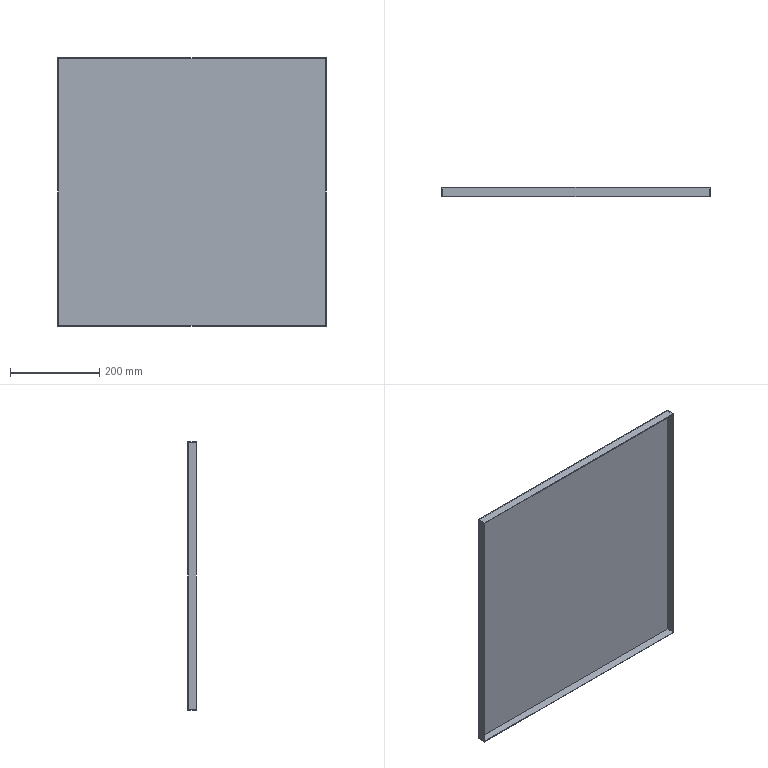Component | SolidWorks | AwningTopPlate-1 | 1 solid | 11 faces | box 600 x 20 x 600 mm | volume 606433 mm3 | plane 11
build123d program:
from build123d import *

# Parameters (mm, degrees)
SKETCH1_W           = 600
SKETCH1_H           = 600
BOSS_EXTRUDE1_DEPTH = 20
SHELL1_T            = -1.5


with BuildPart() as part:
    # Sketch1 → Boss-Extrude1 (new body)
    with BuildSketch(Plane(origin=(0, 0, 0), x_dir=(1, 0, 0), z_dir=(0, 1, 0))):
        Rectangle(SKETCH1_W, SKETCH1_H)
    extrude(amount=BOSS_EXTRUDE1_DEPTH)

    # Shell1
    shell1_openings = [part.faces().sort_by_distance(p)[0] for p in [
        (0, 0, 0),
    ]]
    offset(amount=SHELL1_T, openings=shell1_openings, kind=Kind.INTERSECTION)


solid = part.part

# Placed as in the assembly
solid = solid.moved(Location((0, 1680, 0), (0, 0, 0)))
STEP:
#1=CARTESIAN_POINT('',(11.811,66.142,11.811));
#2=VERTEX_POINT('',#1);
#3=CARTESIAN_POINT('',(11.811,66.142,-11.811));
#4=VERTEX_POINT('',#3);
#5=CARTESIAN_POINT('',(11.811,66.142,-11.811));
#6=DIRECTION('',(0.,0.,-1.));
#7=VECTOR('',#6,39.37);
#8=LINE('',#5,#7);
#9=EDGE_CURVE('',#2,#4,#8,.T.);
#10=ORIENTED_EDGE('',*,*,#9,.T.);
#11=CARTESIAN_POINT('',(11.811,66.929,-11.811));
#12=VERTEX_POINT('',#11);
#13=CARTESIAN_POINT('',(11.811,66.929,-11.811));
#14=DIRECTION('',(0.,-1.,0.));
#15=VECTOR('',#14,39.37);
#16=LINE('',#13,#15);
#17=EDGE_CURVE('',#12,#4,#16,.T.);
#18=ORIENTED_EDGE('',*,*,#17,.F.);
#19=CARTESIAN_POINT('',(11.811,66.929,11.811));
#20=VERTEX_POINT('',#19);
#21=CARTESIAN_POINT('',(11.811,66.929,-11.811));
#22=DIRECTION('',(0.,0.,-1.));
#23=VECTOR('',#22,39.37);
#24=LINE('',#21,#23);
#25=EDGE_CURVE('',#20,#12,#24,.T.);
#26=ORIENTED_EDGE('',*,*,#25,.F.);
#27=CARTESIAN_POINT('',(11.811,66.929,11.811));
#28=DIRECTION('',(0.,-1.,0.));
#29=VECTOR('',#28,39.37);
#30=LINE('',#27,#29);
#31=EDGE_CURVE('',#20,#2,#30,.T.);
#32=ORIENTED_EDGE('',*,*,#31,.T.);
#33=EDGE_LOOP('',(#10,#18,#26,#32));
#34=FACE_OUTER_BOUND('',#33,.T.);
#35=CARTESIAN_POINT('',(11.811,66.929,-11.811));
#36=DIRECTION('',(-1.,0.,0.));
#37=DIRECTION('',(0.,0.,1.));
#38=AXIS2_PLACEMENT_3D('',#35,#36,#37);
#39=PLANE('',#38);
#40=ADVANCED_FACE('',(#34),#39,.F.);
#41=CARTESIAN_POINT('',(-11.811,66.142,-11.811));
#42=VERTEX_POINT('',#41);
#43=CARTESIAN_POINT('',(-11.811,66.142,-11.811));
#44=DIRECTION('',(-1.,0.,0.));
#45=VECTOR('',#44,39.37);
#46=LINE('',#43,#45);
#47=EDGE_CURVE('',#4,#42,#46,.T.);
#48=ORIENTED_EDGE('',*,*,#47,.T.);
#49=CARTESIAN_POINT('',(-11.811,66.929,-11.811));
#50=VERTEX_POINT('',#49);
#51=CARTESIAN_POINT('',(-11.811,66.929,-11.811));
#52=DIRECTION('',(0.,-1.,0.));
#53=VECTOR('',#52,39.37);
#54=LINE('',#51,#53);
#55=EDGE_CURVE('',#50,#42,#54,.T.);
#56=ORIENTED_EDGE('',*,*,#55,.F.);
#57=CARTESIAN_POINT('',(-11.811,66.929,-11.811));
#58=DIRECTION('',(-1.,0.,0.));
#59=VECTOR('',#58,39.37);
#60=LINE('',#57,#59);
#61=EDGE_CURVE('',#12,#50,#60,.T.);
#62=ORIENTED_EDGE('',*,*,#61,.F.);
#63=ORIENTED_EDGE('',*,*,#17,.T.);
#64=EDGE_LOOP('',(#48,#56,#62,#63));
#65=FACE_OUTER_BOUND('',#64,.T.);
#66=CARTESIAN_POINT('',(-11.811,66.929,-11.811));
#67=DIRECTION('',(0.,0.,1.));
#68=DIRECTION('',(1.,0.,0.));
#69=AXIS2_PLACEMENT_3D('',#66,#67,#68);
#70=PLANE('',#69);
#71=ADVANCED_FACE('',(#65),#70,.F.);
#72=CARTESIAN_POINT('',(-11.811,66.142,11.811));
#73=VERTEX_POINT('',#72);
#74=CARTESIAN_POINT('',(-11.811,66.142,-11.811));
#75=DIRECTION('',(0.,0.,1.));
#76=VECTOR('',#75,39.37);
#77=LINE('',#74,#76);
#78=EDGE_CURVE('',#42,#73,#77,.T.);
#79=ORIENTED_EDGE('',*,*,#78,.T.);
#80=CARTESIAN_POINT('',(-11.811,66.929,11.811));
#81=VERTEX_POINT('',#80);
#82=CARTESIAN_POINT('',(-11.811,66.929,11.811));
#83=DIRECTION('',(0.,-1.,0.));
#84=VECTOR('',#83,39.37);
#85=LINE('',#82,#84);
#86=EDGE_CURVE('',#81,#73,#85,.T.);
#87=ORIENTED_EDGE('',*,*,#86,.F.);
#88=CARTESIAN_POINT('',(-11.811,66.929,-11.811));
#89=DIRECTION('',(0.,0.,1.));
#90=VECTOR('',#89,39.37);
#91=LINE('',#88,#90);
#92=EDGE_CURVE('',#50,#81,#91,.T.);
#93=ORIENTED_EDGE('',*,*,#92,.F.);
#94=ORIENTED_EDGE('',*,*,#55,.T.);
#95=EDGE_LOOP('',(#79,#87,#93,#94));
#96=FACE_OUTER_BOUND('',#95,.T.);
#97=CARTESIAN_POINT('',(-11.811,66.929,-11.811));
#98=DIRECTION('',(1.,0.,0.));
#99=DIRECTION('',(0.,0.,-1.));
#100=AXIS2_PLACEMENT_3D('',#97,#98,#99);
#101=PLANE('',#100);
#102=ADVANCED_FACE('',(#96),#101,.F.);
#103=CARTESIAN_POINT('',(-11.811,66.142,11.811));
#104=DIRECTION('',(1.,0.,0.));
#105=VECTOR('',#104,39.37);
#106=LINE('',#103,#105);
#107=EDGE_CURVE('',#73,#2,#106,.T.);
#108=ORIENTED_EDGE('',*,*,#107,.T.);
#109=ORIENTED_EDGE('',*,*,#31,.F.);
#110=CARTESIAN_POINT('',(-11.811,66.929,11.811));
#111=DIRECTION('',(1.,0.,0.));
#112=VECTOR('',#111,39.37);
#113=LINE('',#110,#112);
#114=EDGE_CURVE('',#81,#20,#113,.T.);
#115=ORIENTED_EDGE('',*,*,#114,.F.);
#116=ORIENTED_EDGE('',*,*,#86,.T.);
#117=EDGE_LOOP('',(#108,#109,#115,#116));
#118=FACE_OUTER_BOUND('',#117,.T.);
#119=CARTESIAN_POINT('',(-11.811,66.929,11.811));
#120=DIRECTION('',(0.,0.,-1.));
#121=DIRECTION('',(-1.,0.,0.));
#122=AXIS2_PLACEMENT_3D('',#119,#120,#121);
#123=PLANE('',#122);
#124=ADVANCED_FACE('',(#118),#123,.F.);
#125=ORIENTED_EDGE('',*,*,#25,.T.);
#126=ORIENTED_EDGE('',*,*,#61,.T.);
#127=ORIENTED_EDGE('',*,*,#92,.T.);
#128=ORIENTED_EDGE('',*,*,#114,.T.);
#129=EDGE_LOOP('',(#125,#126,#127,#128));
#130=FACE_OUTER_BOUND('',#129,.T.);
#131=CARTESIAN_POINT('',(0.,66.929,0.));
#132=DIRECTION('',(0.,1.,0.));
#133=DIRECTION('',(0.,0.,1.));
#134=AXIS2_PLACEMENT_3D('',#131,#132,#133);
#135=PLANE('',#134);
#136=ADVANCED_FACE('',(#130),#135,.T.);
#137=CARTESIAN_POINT('',(-11.752,66.142,11.752));
#138=VERTEX_POINT('',#137);
#139=CARTESIAN_POINT('',(11.752,66.142,11.752));
#140=VERTEX_POINT('',#139);
#141=CARTESIAN_POINT('',(-11.811,66.142,11.752));
#142=DIRECTION('',(1.,0.,0.));
#143=VECTOR('',#142,39.37);
#144=LINE('',#141,#143);
#145=EDGE_CURVE('',#138,#140,#144,.T.);
#146=ORIENTED_EDGE('',*,*,#145,.T.);
#147=CARTESIAN_POINT('',(11.752,66.142,-11.752));
#148=VERTEX_POINT('',#147);
#149=CARTESIAN_POINT('',(11.752,66.142,-11.811));
#150=DIRECTION('',(0.,0.,-1.));
#151=VECTOR('',#150,39.37);
#152=LINE('',#149,#151);
#153=EDGE_CURVE('',#140,#148,#152,.T.);
#154=ORIENTED_EDGE('',*,*,#153,.T.);
#155=CARTESIAN_POINT('',(-11.752,66.142,-11.752));
#156=VERTEX_POINT('',#155);
#157=CARTESIAN_POINT('',(-11.811,66.142,-11.752));
#158=DIRECTION('',(-1.,0.,0.));
#159=VECTOR('',#158,39.37);
#160=LINE('',#157,#159);
#161=EDGE_CURVE('',#148,#156,#160,.T.);
#162=ORIENTED_EDGE('',*,*,#161,.T.);
#163=CARTESIAN_POINT('',(-11.752,66.142,-11.811));
#164=DIRECTION('',(0.,0.,1.));
#165=VECTOR('',#164,39.37);
#166=LINE('',#163,#165);
#167=EDGE_CURVE('',#156,#138,#166,.T.);
#168=ORIENTED_EDGE('',*,*,#167,.T.);
#169=EDGE_LOOP('',(#146,#154,#162,#168));
#170=FACE_BOUND('',#169,.T.);
#171=ORIENTED_EDGE('',*,*,#9,.F.);
#172=ORIENTED_EDGE('',*,*,#107,.F.);
#173=ORIENTED_EDGE('',*,*,#78,.F.);
#174=ORIENTED_EDGE('',*,*,#47,.F.);
#175=EDGE_LOOP('',(#171,#172,#173,#174));
#176=FACE_OUTER_BOUND('',#175,.T.);
#177=CARTESIAN_POINT('',(0.,66.142,0.));
#178=DIRECTION('',(0.,1.,0.));
#179=DIRECTION('',(0.,0.,1.));
#180=AXIS2_PLACEMENT_3D('',#177,#178,#179);
#181=PLANE('',#180);
#182=ADVANCED_FACE('',(#170,#176),#181,.F.);
#183=ORIENTED_EDGE('',*,*,#153,.F.);
#184=CARTESIAN_POINT('',(11.752,66.87,11.752));
#185=VERTEX_POINT('',#184);
#186=CARTESIAN_POINT('',(11.752,66.929,11.752));
#187=DIRECTION('',(0.,-1.,0.));
#188=VECTOR('',#187,39.37);
#189=LINE('',#186,#188);
#190=EDGE_CURVE('',#185,#140,#189,.T.);
#191=ORIENTED_EDGE('',*,*,#190,.F.);
#192=CARTESIAN_POINT('',(11.752,66.87,-11.752));
#193=VERTEX_POINT('',#192);
#194=CARTESIAN_POINT('',(11.752,66.87,-11.811));
#195=DIRECTION('',(0.,0.,-1.));
#196=VECTOR('',#195,39.37);
#197=LINE('',#194,#196);
#198=EDGE_CURVE('',#185,#193,#197,.T.);
#199=ORIENTED_EDGE('',*,*,#198,.T.);
#200=CARTESIAN_POINT('',(11.752,66.929,-11.752));
#201=DIRECTION('',(0.,-1.,0.));
#202=VECTOR('',#201,39.37);
#203=LINE('',#200,#202);
#204=EDGE_CURVE('',#193,#148,#203,.T.);
#205=ORIENTED_EDGE('',*,*,#204,.T.);
#206=EDGE_LOOP('',(#183,#191,#199,#205));
#207=FACE_OUTER_BOUND('',#206,.T.);
#208=CARTESIAN_POINT('',(11.752,66.929,-11.811));
#209=DIRECTION('',(-1.,0.,0.));
#210=DIRECTION('',(0.,0.,1.));
#211=AXIS2_PLACEMENT_3D('',#208,#209,#210);
#212=PLANE('',#211);
#213=ADVANCED_FACE('',(#207),#212,.T.);
#214=ORIENTED_EDGE('',*,*,#161,.F.);
#215=ORIENTED_EDGE('',*,*,#204,.F.);
#216=CARTESIAN_POINT('',(-11.752,66.87,-11.752));
#217=VERTEX_POINT('',#216);
#218=CARTESIAN_POINT('',(-11.811,66.87,-11.752));
#219=DIRECTION('',(-1.,0.,0.));
#220=VECTOR('',#219,39.37);
#221=LINE('',#218,#220);
#222=EDGE_CURVE('',#193,#217,#221,.T.);
#223=ORIENTED_EDGE('',*,*,#222,.T.);
#224=CARTESIAN_POINT('',(-11.752,66.929,-11.752));
#225=DIRECTION('',(0.,-1.,0.));
#226=VECTOR('',#225,39.37);
#227=LINE('',#224,#226);
#228=EDGE_CURVE('',#217,#156,#227,.T.);
#229=ORIENTED_EDGE('',*,*,#228,.T.);
#230=EDGE_LOOP('',(#214,#215,#223,#229));
#231=FACE_OUTER_BOUND('',#230,.T.);
#232=CARTESIAN_POINT('',(-11.811,66.929,-11.752));
#233=DIRECTION('',(0.,0.,1.));
#234=DIRECTION('',(1.,0.,0.));
#235=AXIS2_PLACEMENT_3D('',#232,#233,#234);
#236=PLANE('',#235);
#237=ADVANCED_FACE('',(#231),#236,.T.);
#238=ORIENTED_EDGE('',*,*,#167,.F.);
#239=ORIENTED_EDGE('',*,*,#228,.F.);
#240=CARTESIAN_POINT('',(-11.752,66.87,11.752));
#241=VERTEX_POINT('',#240);
#242=CARTESIAN_POINT('',(-11.752,66.87,-11.811));
#243=DIRECTION('',(0.,0.,1.));
#244=VECTOR('',#243,39.37);
#245=LINE('',#242,#244);
#246=EDGE_CURVE('',#217,#241,#245,.T.);
#247=ORIENTED_EDGE('',*,*,#246,.T.);
#248=CARTESIAN_POINT('',(-11.752,66.929,11.752));
#249=DIRECTION('',(0.,-1.,0.));
#250=VECTOR('',#249,39.37);
#251=LINE('',#248,#250);
#252=EDGE_CURVE('',#241,#138,#251,.T.);
#253=ORIENTED_EDGE('',*,*,#252,.T.);
#254=EDGE_LOOP('',(#238,#239,#247,#253));
#255=FACE_OUTER_BOUND('',#254,.T.);
#256=CARTESIAN_POINT('',(-11.752,66.929,-11.811));
#257=DIRECTION('',(1.,0.,0.));
#258=DIRECTION('',(0.,0.,-1.));
#259=AXIS2_PLACEMENT_3D('',#256,#257,#258);
#260=PLANE('',#259);
#261=ADVANCED_FACE('',(#255),#260,.T.);
#262=ORIENTED_EDGE('',*,*,#145,.F.);
#263=ORIENTED_EDGE('',*,*,#252,.F.);
#264=CARTESIAN_POINT('',(-11.811,66.87,11.752));
#265=DIRECTION('',(1.,0.,0.));
#266=VECTOR('',#265,39.37);
#267=LINE('',#264,#266);
#268=EDGE_CURVE('',#241,#185,#267,.T.);
#269=ORIENTED_EDGE('',*,*,#268,.T.);
#270=ORIENTED_EDGE('',*,*,#190,.T.);
#271=EDGE_LOOP('',(#262,#263,#269,#270));
#272=FACE_OUTER_BOUND('',#271,.T.);
#273=CARTESIAN_POINT('',(-11.811,66.929,11.752));
#274=DIRECTION('',(0.,0.,-1.));
#275=DIRECTION('',(-1.,0.,0.));
#276=AXIS2_PLACEMENT_3D('',#273,#274,#275);
#277=PLANE('',#276);
#278=ADVANCED_FACE('',(#272),#277,.T.);
#279=ORIENTED_EDGE('',*,*,#198,.F.);
#280=ORIENTED_EDGE('',*,*,#268,.F.);
#281=ORIENTED_EDGE('',*,*,#246,.F.);
#282=ORIENTED_EDGE('',*,*,#222,.F.);
#283=EDGE_LOOP('',(#279,#280,#281,#282));
#284=FACE_OUTER_BOUND('',#283,.T.);
#285=CARTESIAN_POINT('',(0.,66.87,0.));
#286=DIRECTION('',(0.,1.,0.));
#287=DIRECTION('',(0.,0.,1.));
#288=AXIS2_PLACEMENT_3D('',#285,#286,#287);
#289=PLANE('',#288);
#290=ADVANCED_FACE('',(#284),#289,.F.);
#291=CLOSED_SHELL('',(#40,#71,#102,#124,#136,#182,#213,#237,#261,#278,#290));
#292=MANIFOLD_SOLID_BREP('',#291);
#293=CARTESIAN_POINT('',(0.,0.,0.));
#294=DIRECTION('',(0.,0.,1.));
#295=DIRECTION('',(1.,0.,0.));
#296=AXIS2_PLACEMENT_3D('',#293,#294,#295);
#297=(LENGTH_UNIT()NAMED_UNIT(*)SI_UNIT($,.METRE.));
#298=LENGTH_MEASURE_WITH_UNIT(LENGTH_MEASURE(0.0254),#297);
#299=DIMENSIONAL_EXPONENTS(1.,0.,0.,0.,0.,0.,0.);
#300=(CONVERSION_BASED_UNIT('',#298)LENGTH_UNIT()NAMED_UNIT(#299));
#301=UNCERTAINTY_MEASURE_WITH_UNIT(LENGTH_MEASURE(0.00001),#300,'','');
#302=(NAMED_UNIT(*)PLANE_ANGLE_UNIT()SI_UNIT($,.RADIAN.));
#303=(NAMED_UNIT(*)SI_UNIT($,.STERADIAN.)SOLID_ANGLE_UNIT());
#304=(GEOMETRIC_REPRESENTATION_CONTEXT(3)GLOBAL_UNCERTAINTY_ASSIGNED_CONTEXT((#301))GLOBAL_UNIT_ASSIGNED_CONTEXT((#300,#302,#303))REPRESENTATION_CONTEXT('',''));
#305=ADVANCED_BREP_SHAPE_REPRESENTATION('',(#292,#296),#304);
#306=COLOUR_RGB('',0.7922,0.8196,0.9333);
#307=FILL_AREA_STYLE_COLOUR('',#306);
#308=FILL_AREA_STYLE('',(#307));
#309=SURFACE_STYLE_FILL_AREA(#308);
#310=SURFACE_SIDE_STYLE('',(#309));
#311=SURFACE_STYLE_USAGE(.BOTH.,#310);
#312=PRESENTATION_STYLE_ASSIGNMENT((#311));
#313=STYLED_ITEM('',(#312),#292);
#314=(LENGTH_UNIT()NAMED_UNIT(*)SI_UNIT($,.METRE.));
#315=LENGTH_MEASURE_WITH_UNIT(LENGTH_MEASURE(0.0254),#314);
#316=DIMENSIONAL_EXPONENTS(1.,0.,0.,0.,0.,0.,0.);
#317=(CONVERSION_BASED_UNIT('',#315)LENGTH_UNIT()NAMED_UNIT(#316));
#318=UNCERTAINTY_MEASURE_WITH_UNIT(LENGTH_MEASURE(0.00001),#317,'','');
#319=(NAMED_UNIT(*)PLANE_ANGLE_UNIT()SI_UNIT($,.RADIAN.));
#320=(NAMED_UNIT(*)SI_UNIT($,.STERADIAN.)SOLID_ANGLE_UNIT());
#321=(GEOMETRIC_REPRESENTATION_CONTEXT(3)GLOBAL_UNCERTAINTY_ASSIGNED_CONTEXT((#318))GLOBAL_UNIT_ASSIGNED_CONTEXT((#317,#319,#320))REPRESENTATION_CONTEXT('',''));
#322=MECHANICAL_DESIGN_GEOMETRIC_PRESENTATION_REPRESENTATION('',(#313),#321);
#323=PRESENTATION_LAYER_ASSIGNMENT('','',(#313));